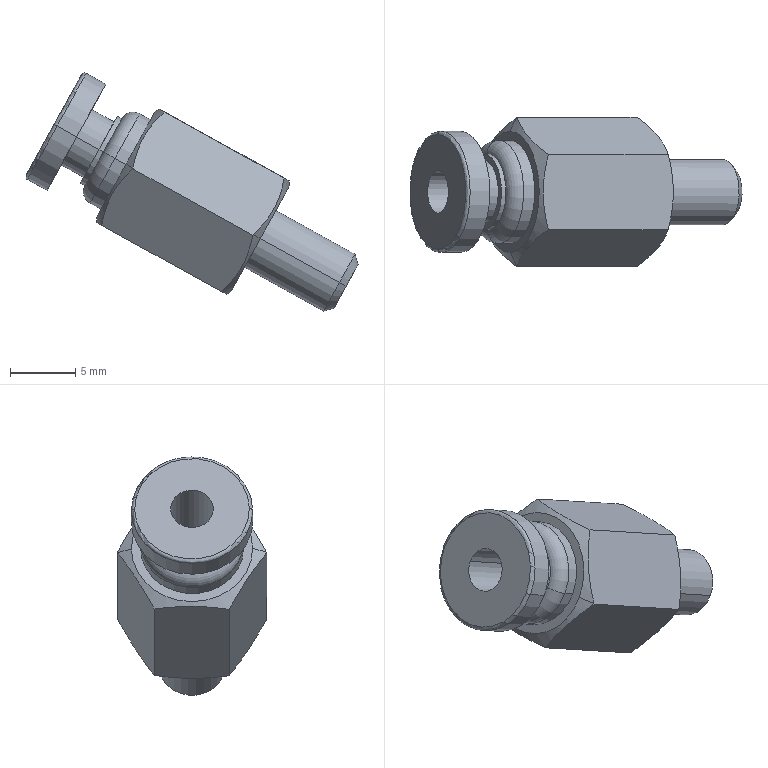Component | SolidWorks | AirSupplyPneumaticQuickConnectorM5-2 | 1 solid | 37 faces | volume 1239 mm3 | cylinder 14 | plane 13 | cone 6 | torus 4 | commonest cylinder face diameters 4.992 x2 7.864 x2 5.864 x2 4.864 x2 9.264 x2 3.264 x2 1.749 x2